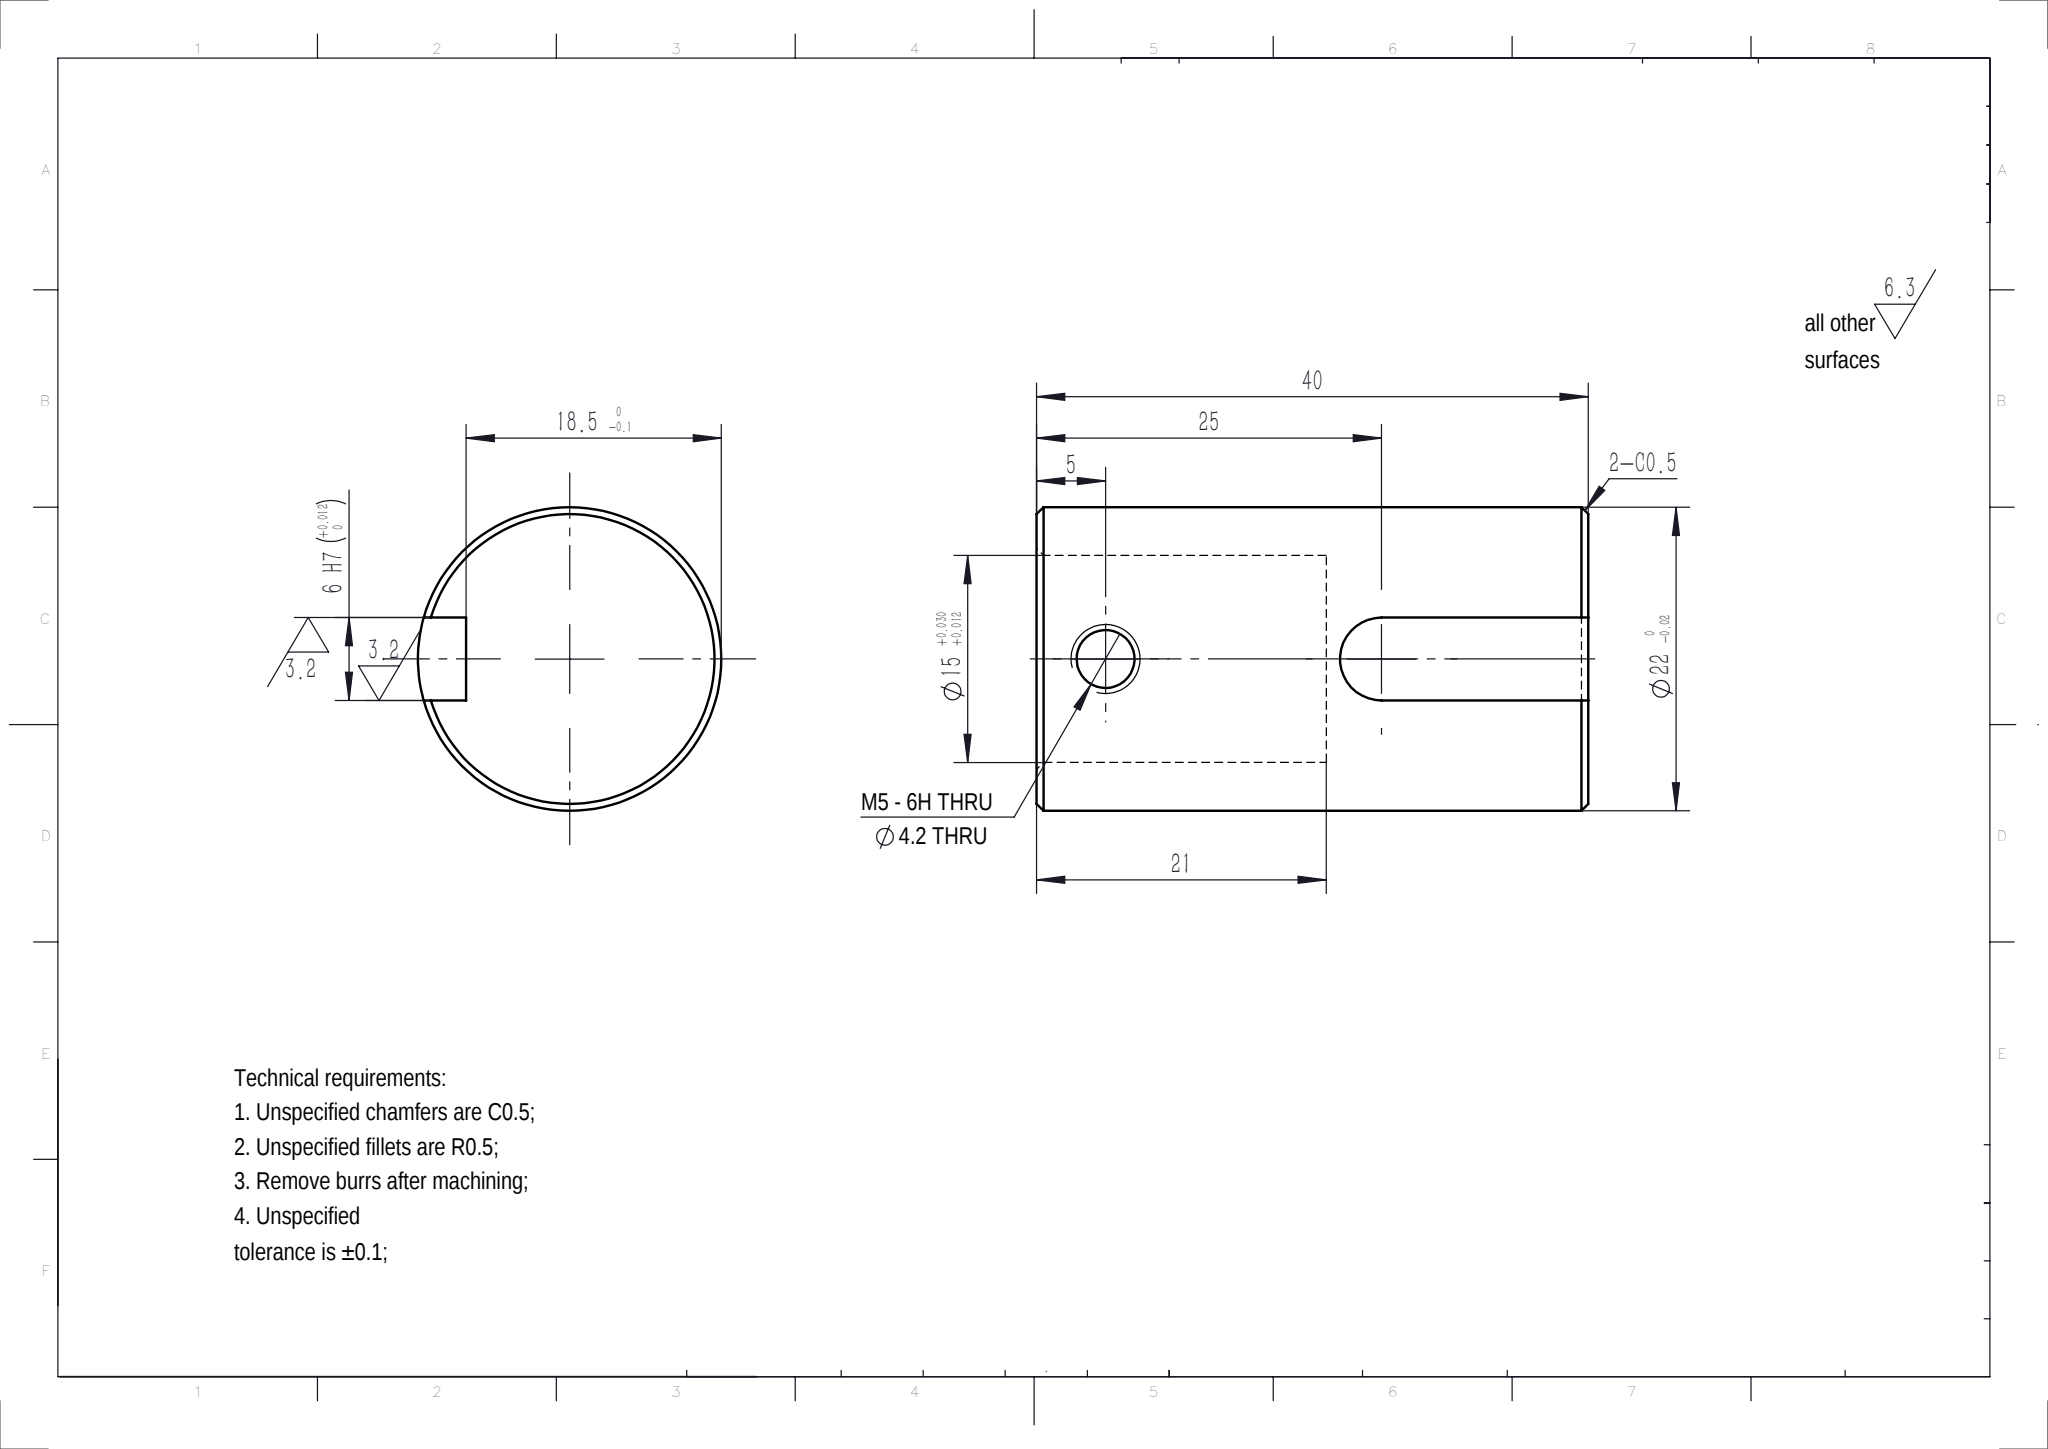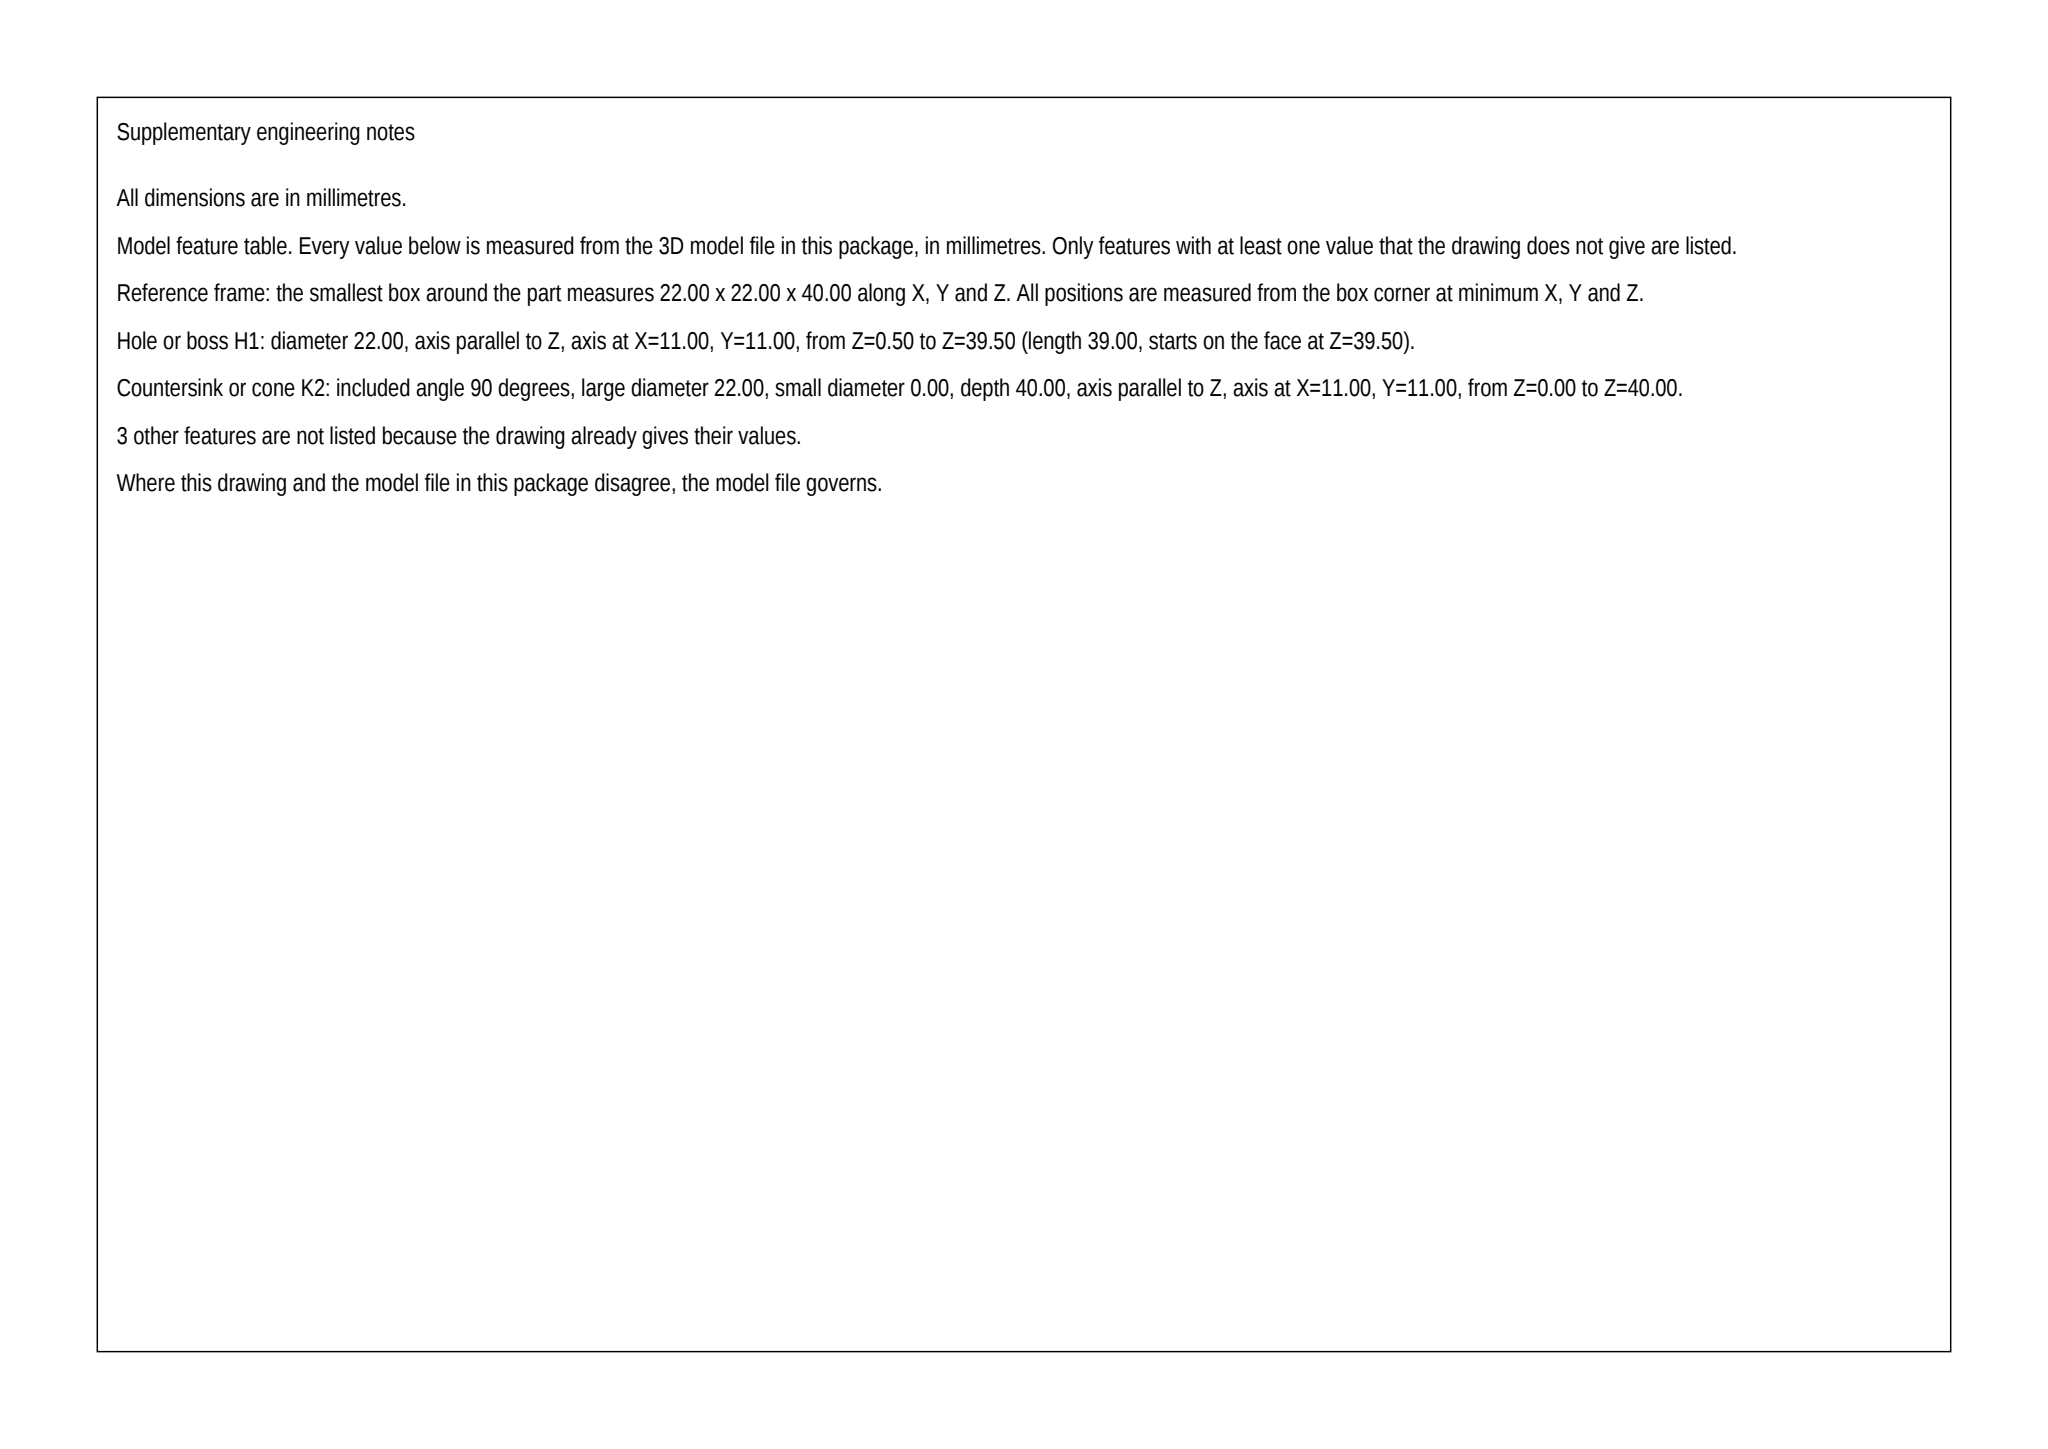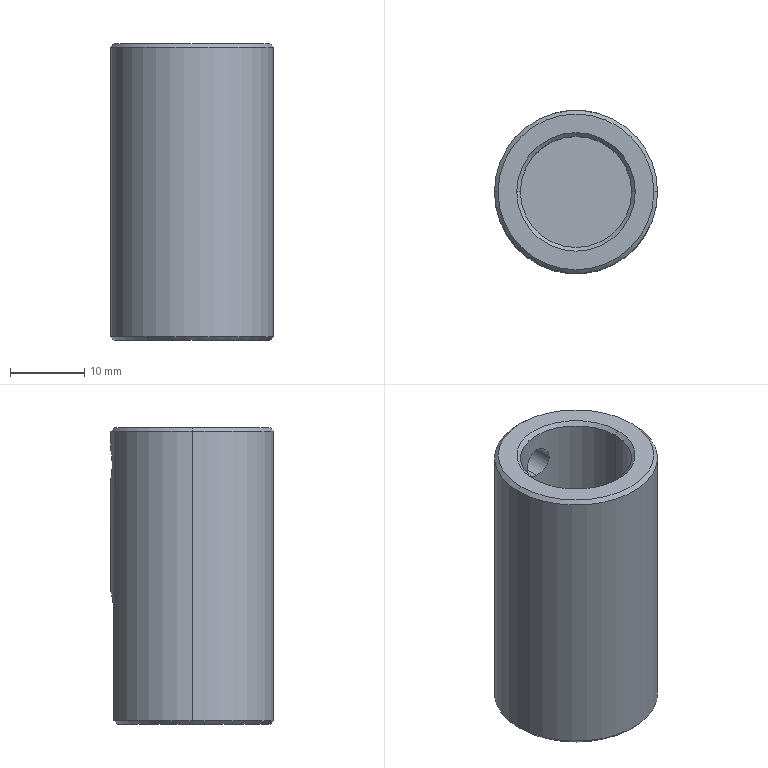Part | SolidWorks | mm | 1 solid | 20 faces | box 22 x 22 x 40 mm | volume 11073 mm3 | cone 7 | cylinder 7 | plane 6 | commonest cylinder face diameters 4.2 x2 15 x2 22 x2 6 x1
build123d program:
from build123d import *

# Parameters (mm, degrees)
SKETCH1_R              = 11
BOSS_EXTRUDE1_DEPTH    = 40
SKETCH2_R              = 7.5
CUT_EXTRUDE1_DEPTH     = 21
M5_TAPPED_HOLE1_REACH  = 44.778
M5_TAPPED_HOLE1_BORE_R = 2.1
CHAMFER1_SIZE          = 0.5
CUT_EXTRUDE2_START     = 7.5
CUT_EXTRUDE2_DEPTH     = 36.419


with BuildPart() as part:
    # Sketch1 → Boss-Extrude1 (new body)
    with BuildSketch(Plane.XY):
        Circle(SKETCH1_R)
    extrude(amount=BOSS_EXTRUDE1_DEPTH)

    # Sketch2 → Cut-Extrude1 (cut)
    with BuildSketch(Plane.XY.offset(40)):
        Circle(SKETCH2_R)
    extrude(amount=-CUT_EXTRUDE1_DEPTH, mode=Mode.SUBTRACT)

    # M5 Tapped Hole1 bore (on position points) → M5 Tapped Hole1 (cut, up to next)
    with BuildSketch(Plane(origin=(0, 11, 35), x_dir=(1, 0, 0), z_dir=(0, 1, 0)), mode=Mode.PRIVATE) as m5_tapped_hole1_sk1:
        Circle(M5_TAPPED_HOLE1_BORE_R)
    m5_tapped_hole1_tool1 = extrude(m5_tapped_hole1_sk1.sketch, amount=-M5_TAPPED_HOLE1_REACH, mode=Mode.PRIVATE) & part.part
    add(m5_tapped_hole1_tool1.solids().sort_by_distance((0, 11, 35))[0], mode=Mode.SUBTRACT)

    # Chamfer1
    chamfer1_edges = [part.edges().sort_by_distance(p)[0] for p in [
        (-11, 0, 0),
        (-11, 0, 40),
        (-7.5, 0, 40),
    ]]
    chamfer(chamfer1_edges, length=CHAMFER1_SIZE)

    # Sketch5 → Cut-Extrude2 (cut, through all)
    with BuildSketch(Plane(origin=(0, 0, 0), x_dir=(1, 0, 0), z_dir=(0, 1, 0)).offset(CUT_EXTRUDE2_START)):
        with BuildLine():
            Line((3, 0), (3, -15))
            ThreePointArc((3, -15), (0, -18), (-3, -15))
            Line((-3, -15), (-3, 0))
            ThreePointArc((-3, 0), (0, 3), (3, 0))
        make_face()
    extrude(amount=CUT_EXTRUDE2_DEPTH, mode=Mode.SUBTRACT)


solid = part.part
STEP:
#1=CARTESIAN_POINT('',(-7.5,0.,39.5));
#2=VERTEX_POINT('',#1);
#3=CARTESIAN_POINT('',(7.5,0.,39.5));
#4=VERTEX_POINT('',#3);
#5=CARTESIAN_POINT('',(0.,0.,39.5));
#6=DIRECTION('',(0.,0.,1.));
#7=DIRECTION('',(1.,0.,0.));
#8=AXIS2_PLACEMENT_3D('',#5,#6,#7);
#9=CIRCLE('',#8,7.5);
#10=EDGE_CURVE('',#2,#4,#9,.T.);
#11=ORIENTED_EDGE('',*,*,#10,.F.);
#12=CARTESIAN_POINT('',(-8.,0.,40.));
#13=VERTEX_POINT('',#12);
#14=CARTESIAN_POINT('',(-7.5,0.,39.5));
#15=DIRECTION('',(-0.7071,0.,0.7071));
#16=VECTOR('',#15,1000.);
#17=LINE('',#14,#16);
#18=EDGE_CURVE('',#2,#13,#17,.T.);
#19=ORIENTED_EDGE('',*,*,#18,.T.);
#20=CARTESIAN_POINT('',(8.,0.,40.));
#21=VERTEX_POINT('',#20);
#22=CARTESIAN_POINT('',(0.,0.,40.));
#23=DIRECTION('',(0.,0.,-1.));
#24=DIRECTION('',(1.,0.,0.));
#25=AXIS2_PLACEMENT_3D('',#22,#23,#24);
#26=CIRCLE('',#25,8.);
#27=EDGE_CURVE('',#21,#13,#26,.T.);
#28=ORIENTED_EDGE('',*,*,#27,.F.);
#29=CARTESIAN_POINT('',(7.5,0.,39.5));
#30=DIRECTION('',(0.7071,0.,0.7071));
#31=VECTOR('',#30,1000.);
#32=LINE('',#29,#31);
#33=EDGE_CURVE('',#4,#21,#32,.T.);
#34=ORIENTED_EDGE('',*,*,#33,.F.);
#35=EDGE_LOOP('',(#11,#19,#28,#34));
#36=FACE_OUTER_BOUND('',#35,.T.);
#37=CARTESIAN_POINT('',(0.,0.,39.5));
#38=DIRECTION('',(0.,0.,1.));
#39=DIRECTION('',(1.,0.,0.));
#40=AXIS2_PLACEMENT_3D('',#37,#38,#39);
#41=CONICAL_SURFACE('',#40,7.5,0.7854);
#42=ADVANCED_FACE('',(#36),#41,.F.);
#43=CARTESIAN_POINT('',(10.5,0.,40.));
#44=VERTEX_POINT('',#43);
#45=CARTESIAN_POINT('',(-10.5,0.,40.));
#46=VERTEX_POINT('',#45);
#47=CARTESIAN_POINT('',(0.,0.,40.));
#48=DIRECTION('',(0.,0.,1.));
#49=DIRECTION('',(1.,0.,0.));
#50=AXIS2_PLACEMENT_3D('',#47,#48,#49);
#51=CIRCLE('',#50,10.5);
#52=EDGE_CURVE('',#44,#46,#51,.T.);
#53=ORIENTED_EDGE('',*,*,#52,.F.);
#54=CARTESIAN_POINT('',(11.,0.,39.5));
#55=VERTEX_POINT('',#54);
#56=CARTESIAN_POINT('',(10.5,0.,40.));
#57=DIRECTION('',(0.7071,0.,-0.7071));
#58=VECTOR('',#57,1000.);
#59=LINE('',#56,#58);
#60=EDGE_CURVE('',#44,#55,#59,.T.);
#61=ORIENTED_EDGE('',*,*,#60,.T.);
#62=CARTESIAN_POINT('',(-11.,0.,39.5));
#63=VERTEX_POINT('',#62);
#64=CARTESIAN_POINT('',(0.,0.,39.5));
#65=DIRECTION('',(0.,0.,-1.));
#66=DIRECTION('',(1.,0.,0.));
#67=AXIS2_PLACEMENT_3D('',#64,#65,#66);
#68=CIRCLE('',#67,11.);
#69=EDGE_CURVE('',#63,#55,#68,.T.);
#70=ORIENTED_EDGE('',*,*,#69,.F.);
#71=CARTESIAN_POINT('',(-10.5,0.,40.));
#72=DIRECTION('',(-0.7071,0.,-0.7071));
#73=VECTOR('',#72,1000.);
#74=LINE('',#71,#73);
#75=EDGE_CURVE('',#46,#63,#74,.T.);
#76=ORIENTED_EDGE('',*,*,#75,.F.);
#77=EDGE_LOOP('',(#53,#61,#70,#76));
#78=FACE_OUTER_BOUND('',#77,.T.);
#79=CARTESIAN_POINT('',(0.,0.,40.));
#80=DIRECTION('',(0.,0.,-1.));
#81=DIRECTION('',(-1.,0.,0.));
#82=AXIS2_PLACEMENT_3D('',#79,#80,#81);
#83=CONICAL_SURFACE('',#82,10.5,0.7854);
#84=ADVANCED_FACE('',(#78),#83,.T.);
#85=CARTESIAN_POINT('',(0.,7.5,32.9));
#86=VERTEX_POINT('',#85);
#87=CARTESIAN_POINT('',(-0.,7.5,37.1));
#88=VERTEX_POINT('',#87);
#89=CARTESIAN_POINT('',(0.,7.5,32.9));
#90=CARTESIAN_POINT('',(-0.2749,7.5,32.9));
#91=CARTESIAN_POINT('',(-0.5525,7.484,32.956));
#92=CARTESIAN_POINT('',(-0.9321,7.443,33.113));
#93=CARTESIAN_POINT('',(-1.055,7.426,33.179));
#94=CARTESIAN_POINT('',(-1.282,7.39,33.331));
#95=CARTESIAN_POINT('',(-1.388,7.371,33.418));
#96=CARTESIAN_POINT('',(-1.581,7.332,33.612));
#97=CARTESIAN_POINT('',(-1.669,7.312,33.719));
#98=CARTESIAN_POINT('',(-1.821,7.276,33.945));
#99=CARTESIAN_POINT('',(-1.886,7.259,34.066));
#100=CARTESIAN_POINT('',(-1.992,7.231,34.321));
#101=CARTESIAN_POINT('',(-2.032,7.219,34.453));
#102=CARTESIAN_POINT('',(-2.086,7.204,34.722));
#103=CARTESIAN_POINT('',(-2.1,7.2,34.861));
#104=CARTESIAN_POINT('',(-2.1,7.2,35.138));
#105=CARTESIAN_POINT('',(-2.086,7.204,35.275));
#106=CARTESIAN_POINT('',(-2.033,7.219,35.545));
#107=CARTESIAN_POINT('',(-1.992,7.231,35.679));
#108=CARTESIAN_POINT('',(-1.834,7.273,36.059));
#109=CARTESIAN_POINT('',(-1.678,7.312,36.292));
#110=CARTESIAN_POINT('',(-1.389,7.371,36.581));
#111=CARTESIAN_POINT('',(-1.283,7.39,36.669));
#112=CARTESIAN_POINT('',(-1.054,7.426,36.821));
#113=CARTESIAN_POINT('',(-0.9341,7.443,36.886));
#114=CARTESIAN_POINT('',(-0.6811,7.47,36.991));
#115=CARTESIAN_POINT('',(-0.5471,7.481,37.032));
#116=CARTESIAN_POINT('',(-0.2768,7.496,37.086));
#117=CARTESIAN_POINT('',(-0.1395,7.5,37.1));
#118=CARTESIAN_POINT('',(-0.,7.5,37.1));
#119=B_SPLINE_CURVE_WITH_KNOTS('',3,(#89,#90,#91,#92,#93,#94,#95,#96,#97,#98,#99,#100,#101,#102,#103,#104,#105,#106,#107,#108,#109,#110,#111,#112,#113,#114,#115,#116,#117,#118),.UNSPECIFIED.,.F.,.F.,(4,2,2,2,2,2,2,2,2,2,2,2,2,2,4),(0.006599,0.007423,0.007836,0.008248,0.00866,0.009073,0.009485,0.009897,0.01031,0.01072,0.01155,0.01196,0.01237,0.01278,0.0132),.UNSPECIFIED.);
#120=EDGE_CURVE('',#86,#88,#119,.T.);
#121=ORIENTED_EDGE('',*,*,#120,.F.);
#122=CARTESIAN_POINT('',(0.,11.,32.9));
#123=VERTEX_POINT('',#122);
#124=CARTESIAN_POINT('',(0.,11.,32.9));
#125=DIRECTION('',(0.,1.,0.));
#126=VECTOR('',#125,1000.);
#127=LINE('',#124,#126);
#128=EDGE_CURVE('',#86,#123,#127,.T.);
#129=ORIENTED_EDGE('',*,*,#128,.T.);
#130=CARTESIAN_POINT('',(0.,11.,37.1));
#131=VERTEX_POINT('',#130);
#132=CARTESIAN_POINT('',(0.,11.,37.1));
#133=CARTESIAN_POINT('',(-0.1391,11.,37.1));
#134=CARTESIAN_POINT('',(-0.2758,10.997,37.086));
#135=CARTESIAN_POINT('',(-0.5447,10.987,37.033));
#136=CARTESIAN_POINT('',(-0.6782,10.98,36.992));
#137=CARTESIAN_POINT('',(-0.9324,10.961,36.887));
#138=CARTESIAN_POINT('',(-1.053,10.95,36.822));
#139=CARTESIAN_POINT('',(-1.281,10.926,36.67));
#140=CARTESIAN_POINT('',(-1.389,10.912,36.581));
#141=CARTESIAN_POINT('',(-1.678,10.873,36.291));
#142=CARTESIAN_POINT('',(-1.835,10.846,36.057));
#143=CARTESIAN_POINT('',(-2.044,10.809,35.552));
#144=CARTESIAN_POINT('',(-2.1,10.798,35.275));
#145=CARTESIAN_POINT('',(-2.1,10.798,34.863));
#146=CARTESIAN_POINT('',(-2.086,10.8,34.724));
#147=CARTESIAN_POINT('',(-2.033,10.811,34.454));
#148=CARTESIAN_POINT('',(-1.993,10.818,34.323));
#149=CARTESIAN_POINT('',(-1.887,10.837,34.069));
#150=CARTESIAN_POINT('',(-1.822,10.848,33.946));
#151=CARTESIAN_POINT('',(-1.67,10.873,33.719));
#152=CARTESIAN_POINT('',(-1.582,10.886,33.613));
#153=CARTESIAN_POINT('',(-1.387,10.913,33.417));
#154=CARTESIAN_POINT('',(-1.281,10.926,33.331));
#155=CARTESIAN_POINT('',(-1.054,10.95,33.179));
#156=CARTESIAN_POINT('',(-0.9313,10.961,33.113));
#157=CARTESIAN_POINT('',(-0.6774,10.98,33.008));
#158=CARTESIAN_POINT('',(-0.5465,10.987,32.968));
#159=CARTESIAN_POINT('',(-0.2766,10.997,32.914));
#160=CARTESIAN_POINT('',(-0.1372,11.,32.9));
#161=CARTESIAN_POINT('',(0.,11.,32.9));
#162=B_SPLINE_CURVE_WITH_KNOTS('',3,(#132,#133,#134,#135,#136,#137,#138,#139,#140,#141,#142,#143,#144,#145,#146,#147,#148,#149,#150,#151,#152,#153,#154,#155,#156,#157,#158,#159,#160,#161),.UNSPECIFIED.,.F.,.F.,(4,2,2,2,2,2,2,2,2,2,2,2,2,2,4),(0.,0.0004113,0.0008226,0.001234,0.001645,0.002468,0.00329,0.003702,0.004113,0.004524,0.004936,0.005347,0.005758,0.006169,0.006581),.UNSPECIFIED.);
#163=EDGE_CURVE('',#131,#123,#162,.T.);
#164=ORIENTED_EDGE('',*,*,#163,.F.);
#165=CARTESIAN_POINT('',(0.,11.,37.1));
#166=DIRECTION('',(0.,1.,0.));
#167=VECTOR('',#166,1000.);
#168=LINE('',#165,#167);
#169=EDGE_CURVE('',#88,#131,#168,.T.);
#170=ORIENTED_EDGE('',*,*,#169,.F.);
#171=EDGE_LOOP('',(#121,#129,#164,#170));
#172=FACE_OUTER_BOUND('',#171,.T.);
#173=CARTESIAN_POINT('',(0.,11.,35.));
#174=DIRECTION('',(0.,1.,0.));
#175=DIRECTION('',(0.,0.,1.));
#176=AXIS2_PLACEMENT_3D('',#173,#174,#175);
#177=CYLINDRICAL_SURFACE('',#176,2.1);
#178=ADVANCED_FACE('',(#172),#177,.F.);
#179=CARTESIAN_POINT('',(-7.5,0.,19.));
#180=VERTEX_POINT('',#179);
#181=CARTESIAN_POINT('',(7.5,0.,19.));
#182=VERTEX_POINT('',#181);
#183=CARTESIAN_POINT('',(0.,0.,19.));
#184=DIRECTION('',(0.,0.,1.));
#185=DIRECTION('',(1.,0.,0.));
#186=AXIS2_PLACEMENT_3D('',#183,#184,#185);
#187=CIRCLE('',#186,7.5);
#188=EDGE_CURVE('',#180,#182,#187,.T.);
#189=ORIENTED_EDGE('',*,*,#188,.F.);
#190=CARTESIAN_POINT('',(-7.5,0.,19.));
#191=DIRECTION('',(0.,0.,1.));
#192=VECTOR('',#191,1000.);
#193=LINE('',#190,#192);
#194=EDGE_CURVE('',#180,#2,#193,.T.);
#195=ORIENTED_EDGE('',*,*,#194,.T.);
#196=ORIENTED_EDGE('',*,*,#10,.T.);
#197=CARTESIAN_POINT('',(7.5,0.,19.));
#198=DIRECTION('',(0.,0.,1.));
#199=VECTOR('',#198,1000.);
#200=LINE('',#197,#199);
#201=EDGE_CURVE('',#182,#4,#200,.T.);
#202=ORIENTED_EDGE('',*,*,#201,.F.);
#203=EDGE_LOOP('',(#189,#195,#196,#202));
#204=FACE_OUTER_BOUND('',#203,.T.);
#205=CARTESIAN_POINT('',(0.,0.,19.));
#206=DIRECTION('',(0.,0.,1.));
#207=DIRECTION('',(1.,0.,0.));
#208=AXIS2_PLACEMENT_3D('',#205,#206,#207);
#209=CYLINDRICAL_SURFACE('',#208,7.5);
#210=ADVANCED_FACE('',(#204),#209,.F.);
#211=CARTESIAN_POINT('',(-10.5,0.,0.));
#212=VERTEX_POINT('',#211);
#213=CARTESIAN_POINT('',(-3.,10.062,0.));
#214=VERTEX_POINT('',#213);
#215=CARTESIAN_POINT('',(0.,0.,0.));
#216=DIRECTION('',(0.,0.,-1.));
#217=DIRECTION('',(1.,0.,0.));
#218=AXIS2_PLACEMENT_3D('',#215,#216,#217);
#219=CIRCLE('',#218,10.5);
#220=EDGE_CURVE('',#212,#214,#219,.T.);
#221=ORIENTED_EDGE('',*,*,#220,.F.);
#222=CARTESIAN_POINT('',(-11.,0.,0.5));
#223=VERTEX_POINT('',#222);
#224=CARTESIAN_POINT('',(-11.,0.,0.5));
#225=DIRECTION('',(-0.7071,0.,0.7071));
#226=VECTOR('',#225,1000.);
#227=LINE('',#224,#226);
#228=EDGE_CURVE('',#212,#223,#227,.T.);
#229=ORIENTED_EDGE('',*,*,#228,.T.);
#230=CARTESIAN_POINT('',(-3.,10.583,0.5));
#231=VERTEX_POINT('',#230);
#232=CARTESIAN_POINT('',(0.,0.,0.5));
#233=DIRECTION('',(0.,0.,1.));
#234=DIRECTION('',(1.,0.,0.));
#235=AXIS2_PLACEMENT_3D('',#232,#233,#234);
#236=CIRCLE('',#235,11.);
#237=EDGE_CURVE('',#231,#223,#236,.T.);
#238=ORIENTED_EDGE('',*,*,#237,.F.);
#239=CARTESIAN_POINT('',(-3.,10.583,0.5));
#240=CARTESIAN_POINT('',(-3.,10.41,0.3332));
#241=CARTESIAN_POINT('',(-3.,10.236,0.1665));
#242=CARTESIAN_POINT('',(-3.,10.062,0.));
#243=B_SPLINE_CURVE_WITH_KNOTS('',3,(#239,#240,#241,#242),.UNSPECIFIED.,.F.,.F.,(4,4),(0.005656,0.006378),.UNSPECIFIED.);
#244=EDGE_CURVE('',#231,#214,#243,.T.);
#245=ORIENTED_EDGE('',*,*,#244,.T.);
#246=EDGE_LOOP('',(#221,#229,#238,#245));
#247=FACE_OUTER_BOUND('',#246,.T.);
#248=CARTESIAN_POINT('',(0.,0.,0.5));
#249=DIRECTION('',(0.,0.,1.));
#250=DIRECTION('',(1.,0.,0.));
#251=AXIS2_PLACEMENT_3D('',#248,#249,#250);
#252=CONICAL_SURFACE('',#251,11.,0.7854);
#253=ADVANCED_FACE('',(#247),#252,.T.);
#254=ORIENTED_EDGE('',*,*,#228,.F.);
#255=CARTESIAN_POINT('',(10.5,0.,0.));
#256=VERTEX_POINT('',#255);
#257=CARTESIAN_POINT('',(0.,0.,0.));
#258=DIRECTION('',(0.,0.,-1.));
#259=DIRECTION('',(1.,0.,0.));
#260=AXIS2_PLACEMENT_3D('',#257,#258,#259);
#261=CIRCLE('',#260,10.5);
#262=EDGE_CURVE('',#256,#212,#261,.T.);
#263=ORIENTED_EDGE('',*,*,#262,.F.);
#264=CARTESIAN_POINT('',(11.,0.,0.5));
#265=VERTEX_POINT('',#264);
#266=CARTESIAN_POINT('',(11.,0.,0.5));
#267=DIRECTION('',(0.7071,0.,0.7071));
#268=VECTOR('',#267,1000.);
#269=LINE('',#266,#268);
#270=EDGE_CURVE('',#256,#265,#269,.T.);
#271=ORIENTED_EDGE('',*,*,#270,.T.);
#272=CARTESIAN_POINT('',(0.,0.,0.5));
#273=DIRECTION('',(0.,0.,1.));
#274=DIRECTION('',(1.,0.,0.));
#275=AXIS2_PLACEMENT_3D('',#272,#273,#274);
#276=CIRCLE('',#275,11.);
#277=EDGE_CURVE('',#223,#265,#276,.T.);
#278=ORIENTED_EDGE('',*,*,#277,.F.);
#279=EDGE_LOOP('',(#254,#263,#271,#278));
#280=FACE_OUTER_BOUND('',#279,.T.);
#281=CARTESIAN_POINT('',(0.,0.,0.5));
#282=DIRECTION('',(0.,0.,1.));
#283=DIRECTION('',(1.,0.,0.));
#284=AXIS2_PLACEMENT_3D('',#281,#282,#283);
#285=CONICAL_SURFACE('',#284,11.,0.7854);
#286=ADVANCED_FACE('',(#280),#285,.T.);
#287=ORIENTED_EDGE('',*,*,#163,.T.);
#288=CARTESIAN_POINT('',(0.,11.,32.9));
#289=CARTESIAN_POINT('',(0.2744,11.,32.9));
#290=CARTESIAN_POINT('',(0.5513,10.989,32.955));
#291=CARTESIAN_POINT('',(0.9305,10.961,33.112));
#292=CARTESIAN_POINT('',(1.053,10.95,33.178));
#293=CARTESIAN_POINT('',(1.282,10.926,33.331));
#294=CARTESIAN_POINT('',(1.387,10.913,33.417));
#295=CARTESIAN_POINT('',(1.581,10.886,33.611));
#296=CARTESIAN_POINT('',(1.669,10.873,33.719));
#297=CARTESIAN_POINT('',(1.822,10.848,33.946));
#298=CARTESIAN_POINT('',(1.886,10.837,34.067));
#299=CARTESIAN_POINT('',(2.045,10.809,34.449));
#300=CARTESIAN_POINT('',(2.1,10.798,34.722));
#301=CARTESIAN_POINT('',(2.1,10.798,35.138));
#302=CARTESIAN_POINT('',(2.087,10.8,35.274));
#303=CARTESIAN_POINT('',(2.033,10.811,35.543));
#304=CARTESIAN_POINT('',(1.993,10.818,35.677));
#305=CARTESIAN_POINT('',(1.887,10.837,35.931));
#306=CARTESIAN_POINT('',(1.823,10.848,36.051));
#307=CARTESIAN_POINT('',(1.671,10.873,36.28));
#308=CARTESIAN_POINT('',(1.582,10.886,36.387));
#309=CARTESIAN_POINT('',(1.293,10.925,36.677));
#310=CARTESIAN_POINT('',(1.059,10.952,36.834));
#311=CARTESIAN_POINT('',(0.6805,10.98,36.991));
#312=CARTESIAN_POINT('',(0.5474,10.987,37.032));
#313=CARTESIAN_POINT('',(0.2763,10.997,37.086));
#314=CARTESIAN_POINT('',(0.1391,11.,37.1));
#315=CARTESIAN_POINT('',(0.,11.,37.1));
#316=B_SPLINE_CURVE_WITH_KNOTS('',3,(#288,#289,#290,#291,#292,#293,#294,#295,#296,#297,#298,#299,#300,#301,#302,#303,#304,#305,#306,#307,#308,#309,#310,#311,#312,#313,#314,#315),.UNSPECIFIED.,.F.,.F.,(4,2,2,2,2,2,2,2,2,2,2,2,2,4),(0.006581,0.007403,0.007814,0.008225,0.008637,0.009048,0.00987,0.01028,0.01069,0.0111,0.01151,0.01234,0.01275,0.01316),.UNSPECIFIED.);
#317=EDGE_CURVE('',#123,#131,#316,.T.);
#318=ORIENTED_EDGE('',*,*,#317,.T.);
#319=EDGE_LOOP('',(#287,#318));
#320=FACE_BOUND('',#319,.T.);
#321=ORIENTED_EDGE('',*,*,#69,.T.);
#322=CARTESIAN_POINT('',(11.,0.,40.));
#323=DIRECTION('',(0.,0.,-1.));
#324=VECTOR('',#323,1000.);
#325=LINE('',#322,#324);
#326=EDGE_CURVE('',#55,#265,#325,.T.);
#327=ORIENTED_EDGE('',*,*,#326,.T.);
#328=CARTESIAN_POINT('',(3.,10.583,0.5));
#329=VERTEX_POINT('',#328);
#330=CARTESIAN_POINT('',(0.,0.,0.5));
#331=DIRECTION('',(0.,0.,1.));
#332=DIRECTION('',(1.,0.,0.));
#333=AXIS2_PLACEMENT_3D('',#330,#331,#332);
#334=CIRCLE('',#333,11.);
#335=EDGE_CURVE('',#265,#329,#334,.T.);
#336=ORIENTED_EDGE('',*,*,#335,.T.);
#337=CARTESIAN_POINT('',(3.,10.583,15.));
#338=VERTEX_POINT('',#337);
#339=CARTESIAN_POINT('',(3.,10.583,40.));
#340=DIRECTION('',(0.,0.,-1.));
#341=VECTOR('',#340,1000.);
#342=LINE('',#339,#341);
#343=EDGE_CURVE('',#338,#329,#342,.T.);
#344=ORIENTED_EDGE('',*,*,#343,.F.);
#345=CARTESIAN_POINT('',(-3.,10.583,15.));
#346=VERTEX_POINT('',#345);
#347=CARTESIAN_POINT('',(-3.,10.583,15.));
#348=CARTESIAN_POINT('',(-3.,10.583,15.199));
#349=CARTESIAN_POINT('',(-2.98,10.589,15.395));
#350=CARTESIAN_POINT('',(-2.904,10.61,15.779));
#351=CARTESIAN_POINT('',(-2.846,10.626,15.97));
#352=CARTESIAN_POINT('',(-2.695,10.665,16.333));
#353=CARTESIAN_POINT('',(-2.603,10.688,16.505));
#354=CARTESIAN_POINT('',(-2.385,10.739,16.83));
#355=CARTESIAN_POINT('',(-2.259,10.766,16.984));
#356=CARTESIAN_POINT('',(-1.984,10.821,17.259));
#357=CARTESIAN_POINT('',(-1.833,10.847,17.383));
#358=CARTESIAN_POINT('',(-1.506,10.898,17.602));
#359=CARTESIAN_POINT('',(-1.333,10.92,17.695));
#360=CARTESIAN_POINT('',(-0.9724,10.958,17.845));
#361=CARTESIAN_POINT('',(-0.7823,10.974,17.903));
#362=CARTESIAN_POINT('',(-0.3947,10.995,17.98));
#363=CARTESIAN_POINT('',(-0.1995,11.,18.));
#364=CARTESIAN_POINT('',(0.1939,11.,18.));
#365=CARTESIAN_POINT('',(0.3937,10.995,17.981));
#366=CARTESIAN_POINT('',(0.7792,10.974,17.904));
#367=CARTESIAN_POINT('',(0.9667,10.959,17.847));
#368=CARTESIAN_POINT('',(1.513,10.902,17.62));
#369=CARTESIAN_POINT('',(1.843,10.848,17.399));
#370=CARTESIAN_POINT('',(2.259,10.766,16.983));
#371=CARTESIAN_POINT('',(2.383,10.739,16.833));
#372=CARTESIAN_POINT('',(2.6,10.689,16.509));
#373=CARTESIAN_POINT('',(2.694,10.665,16.334));
#374=CARTESIAN_POINT('',(2.845,10.626,15.972));
#375=CARTESIAN_POINT('',(2.902,10.61,15.785));
#376=CARTESIAN_POINT('',(2.98,10.589,15.398));
#377=CARTESIAN_POINT('',(3.,10.583,15.199));
#378=CARTESIAN_POINT('',(3.,10.583,15.));
#379=B_SPLINE_CURVE_WITH_KNOTS('',3,(#347,#348,#349,#350,#351,#352,#353,#354,#355,#356,#357,#358,#359,#360,#361,#362,#363,#364,#365,#366,#367,#368,#369,#370,#371,#372,#373,#374,#375,#376,#377,#378),.UNSPECIFIED.,.F.,.F.,(4,2,2,2,2,2,2,2,2,2,2,2,2,2,2,4),(0.,0.0005888,0.001178,0.001766,0.002355,0.002944,0.003533,0.004122,0.004711,0.005299,0.005888,0.007066,0.007655,0.008243,0.008832,0.009421),.UNSPECIFIED.);
#380=EDGE_CURVE('',#346,#338,#379,.T.);
#381=ORIENTED_EDGE('',*,*,#380,.F.);
#382=CARTESIAN_POINT('',(-3.,10.583,40.));
#383=DIRECTION('',(0.,0.,1.));
#384=VECTOR('',#383,1000.);
#385=LINE('',#382,#384);
#386=EDGE_CURVE('',#231,#346,#385,.T.);
#387=ORIENTED_EDGE('',*,*,#386,.F.);
#388=ORIENTED_EDGE('',*,*,#237,.T.);
#389=CARTESIAN_POINT('',(-11.,0.,40.));
#390=DIRECTION('',(0.,0.,-1.));
#391=VECTOR('',#390,1000.);
#392=LINE('',#389,#391);
#393=EDGE_CURVE('',#63,#223,#392,.T.);
#394=ORIENTED_EDGE('',*,*,#393,.F.);
#395=EDGE_LOOP('',(#321,#327,#336,#344,#381,#387,#388,#394));
#396=FACE_OUTER_BOUND('',#395,.T.);
#397=CARTESIAN_POINT('',(0.,0.,40.));
#398=DIRECTION('',(0.,0.,-1.));
#399=DIRECTION('',(-1.,0.,0.));
#400=AXIS2_PLACEMENT_3D('',#397,#398,#399);
#401=CYLINDRICAL_SURFACE('',#400,11.);
#402=ADVANCED_FACE('',(#320,#396),#401,.T.);
#403=ORIENTED_EDGE('',*,*,#326,.F.);
#404=CARTESIAN_POINT('',(0.,0.,39.5));
#405=DIRECTION('',(0.,0.,-1.));
#406=DIRECTION('',(1.,0.,0.));
#407=AXIS2_PLACEMENT_3D('',#404,#405,#406);
#408=CIRCLE('',#407,11.);
#409=EDGE_CURVE('',#55,#63,#408,.T.);
#410=ORIENTED_EDGE('',*,*,#409,.T.);
#411=ORIENTED_EDGE('',*,*,#393,.T.);
#412=ORIENTED_EDGE('',*,*,#277,.T.);
#413=EDGE_LOOP('',(#403,#410,#411,#412));
#414=FACE_OUTER_BOUND('',#413,.T.);
#415=CARTESIAN_POINT('',(0.,0.,40.));
#416=DIRECTION('',(0.,0.,-1.));
#417=DIRECTION('',(-1.,0.,0.));
#418=AXIS2_PLACEMENT_3D('',#415,#416,#417);
#419=CYLINDRICAL_SURFACE('',#418,11.);
#420=ADVANCED_FACE('',(#414),#419,.T.);
#421=CARTESIAN_POINT('',(-3.,7.5,0.));
#422=VERTEX_POINT('',#421);
#423=CARTESIAN_POINT('',(-3.,11.,0.));
#424=DIRECTION('',(0.,-1.,0.));
#425=VECTOR('',#424,1000.);
#426=LINE('',#423,#425);
#427=EDGE_CURVE('',#214,#422,#426,.T.);
#428=ORIENTED_EDGE('',*,*,#427,.T.);
#429=CARTESIAN_POINT('',(3.,7.5,-0.));
#430=VERTEX_POINT('',#429);
#431=CARTESIAN_POINT('',(0.,7.5,0.));
#432=DIRECTION('',(-1.,0.,0.));
#433=VECTOR('',#432,1000.);
#434=LINE('',#431,#433);
#435=EDGE_CURVE('',#430,#422,#434,.T.);
#436=ORIENTED_EDGE('',*,*,#435,.F.);
#437=CARTESIAN_POINT('',(3.,10.062,-0.));
#438=VERTEX_POINT('',#437);
#439=CARTESIAN_POINT('',(3.,11.,-0.));
#440=DIRECTION('',(0.,-1.,0.));
#441=VECTOR('',#440,1000.);
#442=LINE('',#439,#441);
#443=EDGE_CURVE('',#438,#430,#442,.T.);
#444=ORIENTED_EDGE('',*,*,#443,.F.);
#445=CARTESIAN_POINT('',(0.,0.,0.));
#446=DIRECTION('',(0.,0.,-1.));
#447=DIRECTION('',(1.,-0.,0.));
#448=AXIS2_PLACEMENT_3D('',#445,#446,#447);
#449=CIRCLE('',#448,10.5);
#450=EDGE_CURVE('',#438,#256,#449,.T.);
#451=ORIENTED_EDGE('',*,*,#450,.T.);
#452=ORIENTED_EDGE('',*,*,#262,.T.);
#453=ORIENTED_EDGE('',*,*,#220,.T.);
#454=EDGE_LOOP('',(#428,#436,#444,#451,#452,#453));
#455=FACE_OUTER_BOUND('',#454,.T.);
#456=CARTESIAN_POINT('',(0.,0.,0.));
#457=DIRECTION('',(0.,0.,1.));
#458=DIRECTION('',(1.,0.,0.));
#459=AXIS2_PLACEMENT_3D('',#456,#457,#458);
#460=PLANE('',#459);
#461=ADVANCED_FACE('',(#455),#460,.F.);
#462=ORIENTED_EDGE('',*,*,#270,.F.);
#463=ORIENTED_EDGE('',*,*,#450,.F.);
#464=CARTESIAN_POINT('',(3.,10.062,-0.));
#465=CARTESIAN_POINT('',(3.,10.236,0.1665));
#466=CARTESIAN_POINT('',(3.,10.41,0.3332));
#467=CARTESIAN_POINT('',(3.,10.583,0.5));
#468=B_SPLINE_CURVE_WITH_KNOTS('',3,(#464,#465,#466,#467),.UNSPECIFIED.,.F.,.F.,(4,4),(0.006575,0.007297),.UNSPECIFIED.);
#469=EDGE_CURVE('',#438,#329,#468,.T.);
#470=ORIENTED_EDGE('',*,*,#469,.T.);
#471=ORIENTED_EDGE('',*,*,#335,.F.);
#472=EDGE_LOOP('',(#462,#463,#470,#471));
#473=FACE_OUTER_BOUND('',#472,.T.);
#474=CARTESIAN_POINT('',(0.,0.,0.5));
#475=DIRECTION('',(0.,0.,1.));
#476=DIRECTION('',(1.,0.,0.));
#477=AXIS2_PLACEMENT_3D('',#474,#475,#476);
#478=CONICAL_SURFACE('',#477,11.,0.7854);
#479=ADVANCED_FACE('',(#473),#478,.T.);
#480=CARTESIAN_POINT('',(0.,0.,40.));
#481=DIRECTION('',(0.,0.,1.));
#482=DIRECTION('',(1.,0.,0.));
#483=AXIS2_PLACEMENT_3D('',#480,#481,#482);
#484=CIRCLE('',#483,10.5);
#485=EDGE_CURVE('',#46,#44,#484,.T.);
#486=ORIENTED_EDGE('',*,*,#485,.T.);
#487=ORIENTED_EDGE('',*,*,#52,.T.);
#488=EDGE_LOOP('',(#486,#487));
#489=FACE_OUTER_BOUND('',#488,.T.);
#490=ORIENTED_EDGE('',*,*,#27,.T.);
#491=CARTESIAN_POINT('',(0.,0.,40.));
#492=DIRECTION('',(0.,0.,-1.));
#493=DIRECTION('',(1.,0.,0.));
#494=AXIS2_PLACEMENT_3D('',#491,#492,#493);
#495=CIRCLE('',#494,8.);
#496=EDGE_CURVE('',#13,#21,#495,.T.);
#497=ORIENTED_EDGE('',*,*,#496,.T.);
#498=EDGE_LOOP('',(#490,#497));
#499=FACE_BOUND('',#498,.T.);
#500=CARTESIAN_POINT('',(0.,0.,40.));
#501=DIRECTION('',(0.,0.,1.));
#502=DIRECTION('',(1.,0.,0.));
#503=AXIS2_PLACEMENT_3D('',#500,#501,#502);
#504=PLANE('',#503);
#505=ADVANCED_FACE('',(#489,#499),#504,.T.);
#506=ORIENTED_EDGE('',*,*,#194,.F.);
#507=CARTESIAN_POINT('',(0.,0.,19.));
#508=DIRECTION('',(0.,0.,1.));
#509=DIRECTION('',(1.,0.,0.));
#510=AXIS2_PLACEMENT_3D('',#507,#508,#509);
#511=CIRCLE('',#510,7.5);
#512=EDGE_CURVE('',#182,#180,#511,.T.);
#513=ORIENTED_EDGE('',*,*,#512,.F.);
#514=ORIENTED_EDGE('',*,*,#201,.T.);
#515=CARTESIAN_POINT('',(0.,0.,39.5));
#516=DIRECTION('',(0.,0.,1.));
#517=DIRECTION('',(1.,0.,0.));
#518=AXIS2_PLACEMENT_3D('',#515,#516,#517);
#519=CIRCLE('',#518,7.5);
#520=EDGE_CURVE('',#4,#2,#519,.T.);
#521=ORIENTED_EDGE('',*,*,#520,.T.);
#522=EDGE_LOOP('',(#506,#513,#514,#521));
#523=FACE_OUTER_BOUND('',#522,.T.);
#524=CARTESIAN_POINT('',(-0.,7.5,37.1));
#525=CARTESIAN_POINT('',(0.1395,7.5,37.1));
#526=CARTESIAN_POINT('',(0.2765,7.496,37.086));
#527=CARTESIAN_POINT('',(0.5459,7.481,37.032));
#528=CARTESIAN_POINT('',(0.6797,7.47,36.992));
#529=CARTESIAN_POINT('',(0.9337,7.443,36.886));
#530=CARTESIAN_POINT('',(1.054,7.426,36.821));
#531=CARTESIAN_POINT('',(1.282,7.391,36.669));
#532=CARTESIAN_POINT('',(1.389,7.371,36.581));
#533=CARTESIAN_POINT('',(1.678,7.313,36.292));
#534=CARTESIAN_POINT('',(1.834,7.273,36.059));
#535=CARTESIAN_POINT('',(1.992,7.231,35.68));
#536=CARTESIAN_POINT('',(2.032,7.219,35.547));
#537=CARTESIAN_POINT('',(2.086,7.204,35.275));
#538=CARTESIAN_POINT('',(2.1,7.2,35.139));
#539=CARTESIAN_POINT('',(2.1,7.2,34.863));
#540=CARTESIAN_POINT('',(2.086,7.204,34.723));
#541=CARTESIAN_POINT('',(2.032,7.219,34.453));
#542=CARTESIAN_POINT('',(1.992,7.231,34.322));
#543=CARTESIAN_POINT('',(1.833,7.273,33.939));
#544=CARTESIAN_POINT('',(1.679,7.312,33.709));
#545=CARTESIAN_POINT('',(1.387,7.371,33.418));
#546=CARTESIAN_POINT('',(1.282,7.39,33.331));
#547=CARTESIAN_POINT('',(1.055,7.426,33.179));
#548=CARTESIAN_POINT('',(0.9321,7.443,33.113));
#549=CARTESIAN_POINT('',(0.6788,7.47,33.008));
#550=CARTESIAN_POINT('',(0.5478,7.481,32.968));
#551=CARTESIAN_POINT('',(0.2769,7.496,32.914));
#552=CARTESIAN_POINT('',(0.1375,7.5,32.9));
#553=CARTESIAN_POINT('',(0.,7.5,32.9));
#554=B_SPLINE_CURVE_WITH_KNOTS('',3,(#524,#525,#526,#527,#528,#529,#530,#531,#532,#533,#534,#535,#536,#537,#538,#539,#540,#541,#542,#543,#544,#545,#546,#547,#548,#549,#550,#551,#552,#553),.UNSPECIFIED.,.F.,.F.,(4,2,2,2,2,2,2,2,2,2,2,2,2,2,4),(0.,0.0004124,0.0008248,0.001237,0.00165,0.002475,0.002887,0.003299,0.003712,0.004124,0.004949,0.005361,0.005774,0.006186,0.006599),.UNSPECIFIED.);
#555=EDGE_CURVE('',#88,#86,#554,.T.);
#556=ORIENTED_EDGE('',*,*,#555,.T.);
#557=ORIENTED_EDGE('',*,*,#120,.T.);
#558=EDGE_LOOP('',(#556,#557));
#559=FACE_BOUND('',#558,.T.);
#560=CARTESIAN_POINT('',(0.,0.,19.));
#561=DIRECTION('',(0.,0.,1.));
#562=DIRECTION('',(1.,0.,0.));
#563=AXIS2_PLACEMENT_3D('',#560,#561,#562);
#564=CYLINDRICAL_SURFACE('',#563,7.5);
#565=ADVANCED_FACE('',(#523,#559),#564,.F.);
#566=ORIENTED_EDGE('',*,*,#512,.T.);
#567=ORIENTED_EDGE('',*,*,#188,.T.);
#568=EDGE_LOOP('',(#566,#567));
#569=FACE_OUTER_BOUND('',#568,.T.);
#570=CARTESIAN_POINT('',(0.,0.,19.));
#571=DIRECTION('',(0.,0.,1.));
#572=DIRECTION('',(1.,0.,0.));
#573=AXIS2_PLACEMENT_3D('',#570,#571,#572);
#574=PLANE('',#573);
#575=ADVANCED_FACE('',(#569),#574,.T.);
#576=ORIENTED_EDGE('',*,*,#128,.F.);
#577=ORIENTED_EDGE('',*,*,#555,.F.);
#578=ORIENTED_EDGE('',*,*,#169,.T.);
#579=ORIENTED_EDGE('',*,*,#317,.F.);
#580=EDGE_LOOP('',(#576,#577,#578,#579));
#581=FACE_OUTER_BOUND('',#580,.T.);
#582=CARTESIAN_POINT('',(0.,11.,35.));
#583=DIRECTION('',(0.,1.,0.));
#584=DIRECTION('',(0.,0.,1.));
#585=AXIS2_PLACEMENT_3D('',#582,#583,#584);
#586=CYLINDRICAL_SURFACE('',#585,2.1);
#587=ADVANCED_FACE('',(#581),#586,.F.);
#588=ORIENTED_EDGE('',*,*,#60,.F.);
#589=ORIENTED_EDGE('',*,*,#485,.F.);
#590=ORIENTED_EDGE('',*,*,#75,.T.);
#591=ORIENTED_EDGE('',*,*,#409,.F.);
#592=EDGE_LOOP('',(#588,#589,#590,#591));
#593=FACE_OUTER_BOUND('',#592,.T.);
#594=CARTESIAN_POINT('',(0.,0.,40.));
#595=DIRECTION('',(0.,0.,-1.));
#596=DIRECTION('',(-1.,0.,0.));
#597=AXIS2_PLACEMENT_3D('',#594,#595,#596);
#598=CONICAL_SURFACE('',#597,10.5,0.7854);
#599=ADVANCED_FACE('',(#593),#598,.T.);
#600=ORIENTED_EDGE('',*,*,#18,.F.);
#601=ORIENTED_EDGE('',*,*,#520,.F.);
#602=ORIENTED_EDGE('',*,*,#33,.T.);
#603=ORIENTED_EDGE('',*,*,#496,.F.);
#604=EDGE_LOOP('',(#600,#601,#602,#603));
#605=FACE_OUTER_BOUND('',#604,.T.);
#606=CARTESIAN_POINT('',(0.,0.,39.5));
#607=DIRECTION('',(0.,0.,1.));
#608=DIRECTION('',(1.,0.,0.));
#609=AXIS2_PLACEMENT_3D('',#606,#607,#608);
#610=CONICAL_SURFACE('',#609,7.5,0.7854);
#611=ADVANCED_FACE('',(#605),#610,.F.);
#612=CARTESIAN_POINT('',(-3.,7.5,15.));
#613=VERTEX_POINT('',#612);
#614=CARTESIAN_POINT('',(-3.,11.,15.));
#615=DIRECTION('',(0.,-1.,0.));
#616=VECTOR('',#615,1000.);
#617=LINE('',#614,#616);
#618=EDGE_CURVE('',#346,#613,#617,.T.);
#619=ORIENTED_EDGE('',*,*,#618,.F.);
#620=ORIENTED_EDGE('',*,*,#380,.T.);
#621=CARTESIAN_POINT('',(3.,7.5,15.));
#622=VERTEX_POINT('',#621);
#623=CARTESIAN_POINT('',(3.,11.,15.));
#624=DIRECTION('',(0.,-1.,0.));
#625=VECTOR('',#624,1000.);
#626=LINE('',#623,#625);
#627=EDGE_CURVE('',#338,#622,#626,.T.);
#628=ORIENTED_EDGE('',*,*,#627,.T.);
#629=CARTESIAN_POINT('',(0.,7.5,15.));
#630=DIRECTION('',(0.,1.,0.));
#631=DIRECTION('',(0.,0.,1.));
#632=AXIS2_PLACEMENT_3D('',#629,#630,#631);
#633=CIRCLE('',#632,3.);
#634=EDGE_CURVE('',#613,#622,#633,.T.);
#635=ORIENTED_EDGE('',*,*,#634,.F.);
#636=EDGE_LOOP('',(#619,#620,#628,#635));
#637=FACE_OUTER_BOUND('',#636,.T.);
#638=CARTESIAN_POINT('',(0.,11.,15.));
#639=DIRECTION('',(0.,-1.,0.));
#640=DIRECTION('',(0.,0.,-1.));
#641=AXIS2_PLACEMENT_3D('',#638,#639,#640);
#642=CYLINDRICAL_SURFACE('',#641,3.);
#643=ADVANCED_FACE('',(#637),#642,.F.);
#644=ORIENTED_EDGE('',*,*,#435,.T.);
#645=CARTESIAN_POINT('',(-3.,7.5,0.));
#646=DIRECTION('',(0.,0.,1.));
#647=VECTOR('',#646,1000.);
#648=LINE('',#645,#647);
#649=EDGE_CURVE('',#422,#613,#648,.T.);
#650=ORIENTED_EDGE('',*,*,#649,.T.);
#651=ORIENTED_EDGE('',*,*,#634,.T.);
#652=CARTESIAN_POINT('',(3.,7.5,-0.));
#653=DIRECTION('',(-0.,0.,-1.));
#654=VECTOR('',#653,1000.);
#655=LINE('',#652,#654);
#656=EDGE_CURVE('',#622,#430,#655,.T.);
#657=ORIENTED_EDGE('',*,*,#656,.T.);
#658=EDGE_LOOP('',(#644,#650,#651,#657));
#659=FACE_OUTER_BOUND('',#658,.T.);
#660=CARTESIAN_POINT('',(0.,7.5,0.));
#661=DIRECTION('',(0.,1.,0.));
#662=DIRECTION('',(0.,0.,1.));
#663=AXIS2_PLACEMENT_3D('',#660,#661,#662);
#664=PLANE('',#663);
#665=ADVANCED_FACE('',(#659),#664,.T.);
#666=ORIENTED_EDGE('',*,*,#386,.T.);
#667=ORIENTED_EDGE('',*,*,#618,.T.);
#668=ORIENTED_EDGE('',*,*,#649,.F.);
#669=ORIENTED_EDGE('',*,*,#427,.F.);
#670=ORIENTED_EDGE('',*,*,#244,.F.);
#671=EDGE_LOOP('',(#666,#667,#668,#669,#670));
#672=FACE_OUTER_BOUND('',#671,.T.);
#673=CARTESIAN_POINT('',(-3.,11.,0.));
#674=DIRECTION('',(1.,0.,-0.));
#675=DIRECTION('',(-0.,0.,-1.));
#676=AXIS2_PLACEMENT_3D('',#673,#674,#675);
#677=PLANE('',#676);
#678=ADVANCED_FACE('',(#672),#677,.T.);
#679=ORIENTED_EDGE('',*,*,#343,.T.);
#680=ORIENTED_EDGE('',*,*,#469,.F.);
#681=ORIENTED_EDGE('',*,*,#443,.T.);
#682=ORIENTED_EDGE('',*,*,#656,.F.);
#683=ORIENTED_EDGE('',*,*,#627,.F.);
#684=EDGE_LOOP('',(#679,#680,#681,#682,#683));
#685=FACE_OUTER_BOUND('',#684,.T.);
#686=CARTESIAN_POINT('',(3.,11.,-0.));
#687=DIRECTION('',(-1.,0.,0.));
#688=DIRECTION('',(0.,0.,1.));
#689=AXIS2_PLACEMENT_3D('',#686,#687,#688);
#690=PLANE('',#689);
#691=ADVANCED_FACE('',(#685),#690,.T.);
#692=CLOSED_SHELL('',(#42,#84,#178,#210,#253,#286,#402,#420,#461,#479,#505,#565,#575,#587,#599,#611,#643,#665,#678,#691));
#693=MANIFOLD_SOLID_BREP('',#692);
#694=CARTESIAN_POINT('',(0.,0.,0.));
#695=DIRECTION('',(0.,0.,1.));
#696=DIRECTION('',(1.,0.,0.));
#697=AXIS2_PLACEMENT_3D('',#694,#695,#696);
#698=(LENGTH_UNIT()NAMED_UNIT(*)SI_UNIT(.MILLI.,.METRE.));
#699=UNCERTAINTY_MEASURE_WITH_UNIT(LENGTH_MEASURE(0.00001),#698,'','');
#700=(NAMED_UNIT(*)PLANE_ANGLE_UNIT()SI_UNIT($,.RADIAN.));
#701=(NAMED_UNIT(*)SI_UNIT($,.STERADIAN.)SOLID_ANGLE_UNIT());
#702=(GEOMETRIC_REPRESENTATION_CONTEXT(3)GLOBAL_UNCERTAINTY_ASSIGNED_CONTEXT((#699))GLOBAL_UNIT_ASSIGNED_CONTEXT((#698,#700,#701))REPRESENTATION_CONTEXT('',''));
#703=ADVANCED_BREP_SHAPE_REPRESENTATION('',(#693,#697),#702);